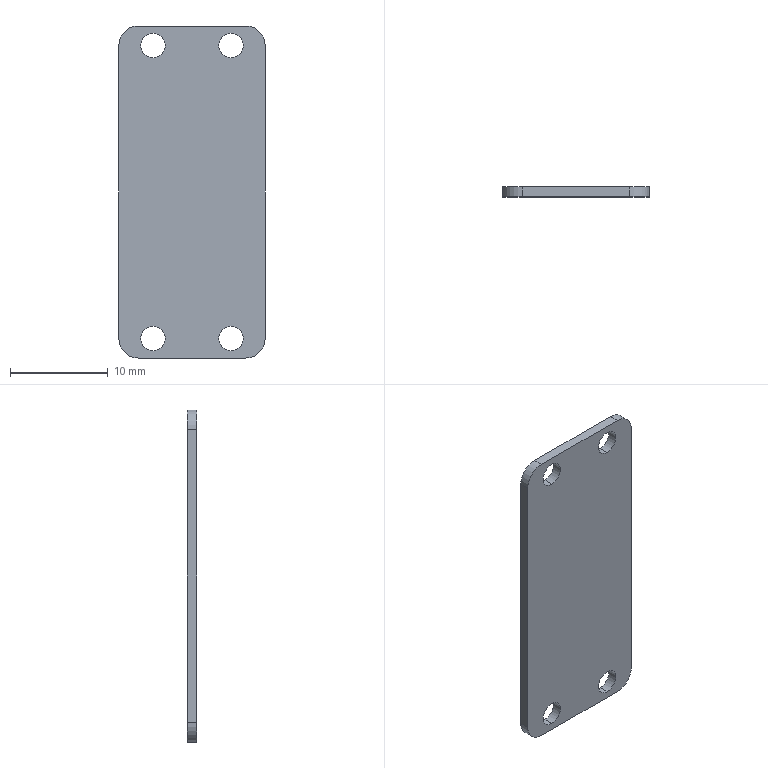CAM job | NX | mm | 3-axis | 1 set-up | 200 operations | part box 15 x 1 x 34
set-up 1
1. Cylinder Milling | Mill Mill5 LX-D1.5 | CYLINDER_MILLING_1 | path 297.004 mm | 0.1342 min
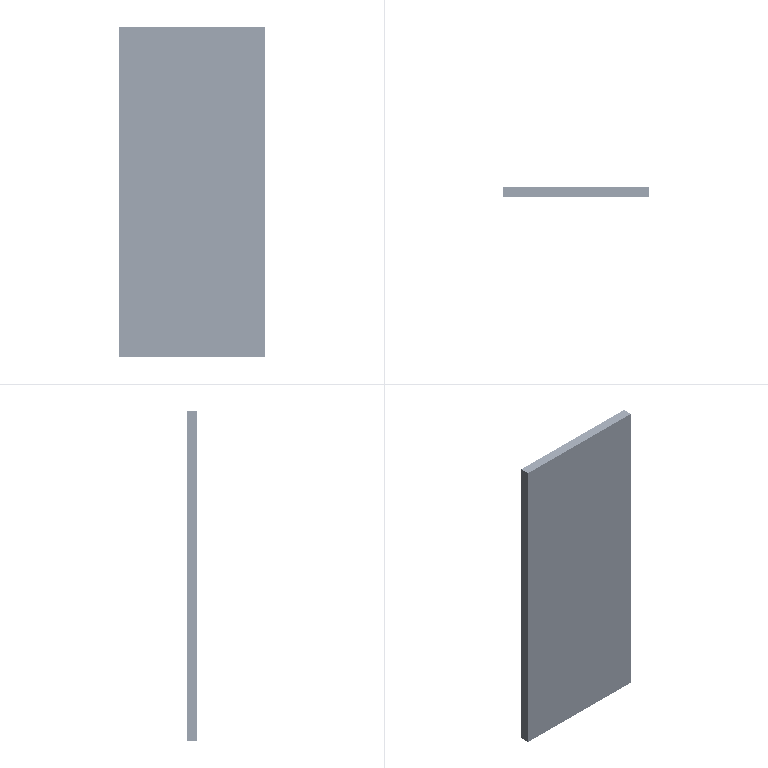2. Volume Based 2.5D Milling | Mill Mill5 LX-D1.5 | VOLUME_BASED_2.5D_MILLING_2 | path 646.751 mm | 0.2089 min
3. Cylinder Milling | Mill Mill5 LX-D1.5 | CYLINDER_MILLING_3 | path 297.004 mm | 0.1342 min
4. Volume Based 2.5D Milling | Mill Mill5 LX-D1.5 | VOLUME_BASED_2.5D_MILLING_4 | path 646.751 mm | 0.2089 min
5. Cylinder Milling | Mill Mill5 LX-D1.5 | CYLINDER_MILLING_5 | path 297.004 mm | 0.1342 min
6. Volume Based 2.5D Milling | Mill Mill5 LX-D1.5 | VOLUME_BASED_2.5D_MILLING_6 | path 646.751 mm | 0.2089 min
7. Cylinder Milling | Mill Mill5 LX-D1.5 | CYLINDER_MILLING_7 | path 297.004 mm | 0.1342 min
8. Volume Based 2.5D Milling | Mill Mill5 LX-D1.5 | VOLUME_BASED_2.5D_MILLING_8 | path 646.751 mm | 0.2089 min
9. Cylinder Milling | Mill Mill5 LX-D1.5 | CYLINDER_MILLING_9 | path 297.004 mm | 0.1342 min
10. Volume Based 2.5D Milling | Mill Mill5 LX-D1.5 | VOLUME_BASED_2.5D_MILLING_10 | path 646.751 mm | 0.2089 min
11. Cylinder Milling | Mill Mill5 LX-D1.5 | CYLINDER_MILLING_11 | path 297.004 mm | 0.1342 min
12. Volume Based 2.5D Milling | Mill Mill5 LX-D1.5 | VOLUME_BASED_2.5D_MILLING_12 | path 646.751 mm | 0.2089 min
13. Cylinder Milling | Mill Mill5 LX-D1.5 | CYLINDER_MILLING_13 | path 297.004 mm | 0.1342 min
14. Volume Based 2.5D Milling | Mill Mill5 LX-D1.5 | VOLUME_BASED_2.5D_MILLING_14 | path 646.751 mm | 0.2089 min
15. Cylinder Milling | Mill Mill5 LX-D1.5 | CYLINDER_MILLING_15 | path 297.004 mm | 0.1342 min
16. Volume Based 2.5D Milling | Mill Mill5 LX-D1.5 | VOLUME_BASED_2.5D_MILLING_16 | path 646.751 mm | 0.2089 min
17. Cylinder Milling | Mill Mill5 LX-D1.5 | CYLINDER_MILLING_17 | path 297.004 mm | 0.1342 min
18. Volume Based 2.5D Milling | Mill Mill5 LX-D1.5 | VOLUME_BASED_2.5D_MILLING_18 | path 646.751 mm | 0.2089 min
19. Cylinder Milling | Mill Mill5 LX-D1.5 | CYLINDER_MILLING_19 | path 297.004 mm | 0.1342 min
20. Volume Based 2.5D Milling | Mill Mill5 LX-D1.5 | VOLUME_BASED_2.5D_MILLING_20 | path 646.751 mm | 0.2089 min
21. Cylinder Milling | Mill Mill5 LX-D1.5 | CYLINDER_MILLING_21 | path 297.004 mm | 0.1342 min
22. Volume Based 2.5D Milling | Mill Mill5 LX-D1.5 | VOLUME_BASED_2.5D_MILLING_22 | path 646.751 mm | 0.2089 min
23. Cylinder Milling | Mill Mill5 LX-D1.5 | CYLINDER_MILLING_23 | path 297.004 mm | 0.1342 min
24. Volume Based 2.5D Milling | Mill Mill5 LX-D1.5 | VOLUME_BASED_2.5D_MILLING_24 | path 646.751 mm | 0.2089 min
25. Cylinder Milling | Mill Mill5 LX-D1.5 | CYLINDER_MILLING_25 | path 297.004 mm | 0.1342 min
26. Volume Based 2.5D Milling | Mill Mill5 LX-D1.5 | VOLUME_BASED_2.5D_MILLING_26 | path 646.751 mm | 0.2089 min
27. Cylinder Milling | Mill Mill5 LX-D1.5 | CYLINDER_MILLING_27 | path 297.004 mm | 0.1342 min
28. Volume Based 2.5D Milling | Mill Mill5 LX-D1.5 | VOLUME_BASED_2.5D_MILLING_28 | path 646.751 mm | 0.2089 min
29. Cylinder Milling | Mill Mill5 LX-D1.5 | CYLINDER_MILLING_29 | path 297.004 mm | 0.1342 min
30. Volume Based 2.5D Milling | Mill Mill5 LX-D1.5 | VOLUME_BASED_2.5D_MILLING_30 | path 646.751 mm | 0.2089 min
31. Cylinder Milling | Mill Mill5 LX-D1.5 | CYLINDER_MILLING_31 | path 297.004 mm | 0.1342 min
32. Volume Based 2.5D Milling | Mill Mill5 LX-D1.5 | VOLUME_BASED_2.5D_MILLING_32 | path 646.751 mm | 0.2089 min
33. Cylinder Milling | Mill Mill5 LX-D1.5 | CYLINDER_MILLING_33 | path 297.004 mm | 0.1342 min
34. Volume Based 2.5D Milling | Mill Mill5 LX-D1.5 | VOLUME_BASED_2.5D_MILLING_34 | path 646.751 mm | 0.2089 min
35. Cylinder Milling | Mill Mill5 LX-D1.5 | CYLINDER_MILLING_35 | path 297.004 mm | 0.1342 min
36. Volume Based 2.5D Milling | Mill Mill5 LX-D1.5 | VOLUME_BASED_2.5D_MILLING_36 | path 646.751 mm | 0.2089 min
37. Cylinder Milling | Mill Mill5 LX-D1.5 | CYLINDER_MILLING_37 | path 297.004 mm | 0.1342 min
38. Volume Based 2.5D Milling | Mill Mill5 LX-D1.5 | VOLUME_BASED_2.5D_MILLING_38 | path 646.751 mm | 0.2089 min
39. Cylinder Milling | Mill Mill5 LX-D1.5 | CYLINDER_MILLING_39 | path 297.004 mm | 0.1342 min
40. Volume Based 2.5D Milling | Mill Mill5 LX-D1.5 | VOLUME_BASED_2.5D_MILLING_40 | path 646.751 mm | 0.2089 min
41. Cylinder Milling | Mill Mill5 LX-D1.5 | CYLINDER_MILLING_41 | path 297.004 mm | 0.1342 min
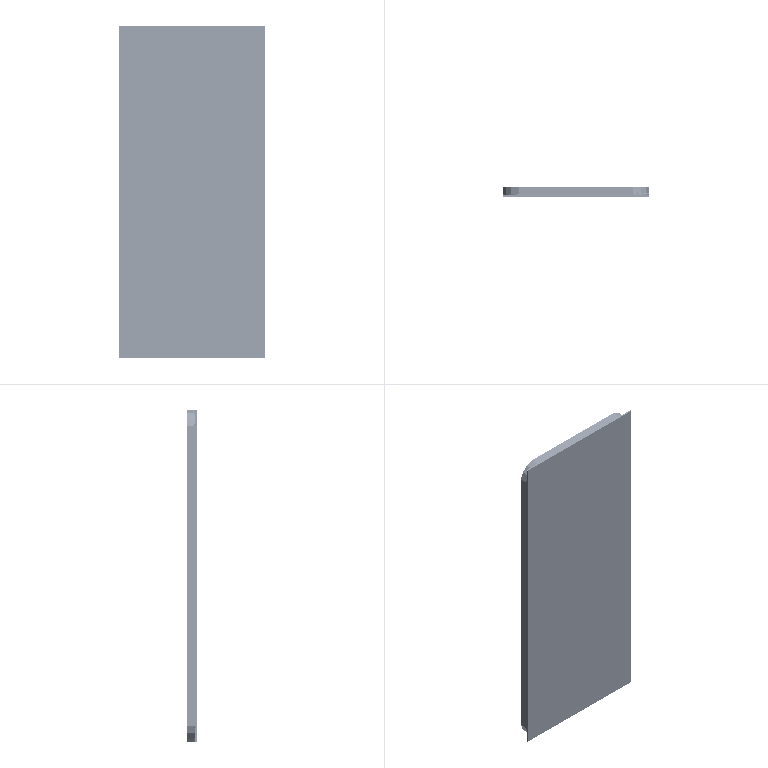42. Volume Based 2.5D Milling | Mill Mill5 LX-D1.5 | VOLUME_BASED_2.5D_MILLING_42 | path 646.751 mm | 0.2089 min
43. Cylinder Milling | Mill Mill5 LX-D1.5 | CYLINDER_MILLING_43 | path 297.004 mm | 0.1342 min
44. Volume Based 2.5D Milling | Mill Mill5 LX-D1.5 | VOLUME_BASED_2.5D_MILLING_44 | path 646.751 mm | 0.2089 min
45. Cylinder Milling | Mill Mill5 LX-D1.5 | CYLINDER_MILLING_45 | path 297.004 mm | 0.1342 min
46. Volume Based 2.5D Milling | Mill Mill5 LX-D1.5 | VOLUME_BASED_2.5D_MILLING_46 | path 646.751 mm | 0.2089 min
47. Cylinder Milling | Mill Mill5 LX-D1.5 | CYLINDER_MILLING_47 | path 297.004 mm | 0.1342 min
48. Volume Based 2.5D Milling | Mill Mill5 LX-D1.5 | VOLUME_BASED_2.5D_MILLING_48 | path 646.751 mm | 0.2089 min
49. Cylinder Milling | Mill Mill5 LX-D1.5 | CYLINDER_MILLING_49 | path 297.004 mm | 0.1342 min
50. Volume Based 2.5D Milling | Mill Mill5 LX-D1.5 | VOLUME_BASED_2.5D_MILLING_50 | path 646.751 mm | 0.2089 min
51. Cylinder Milling | Mill Mill5 LX-D1.5 | CYLINDER_MILLING_51 | path 297.004 mm | 0.1342 min
52. Volume Based 2.5D Milling | Mill Mill5 LX-D1.5 | VOLUME_BASED_2.5D_MILLING_52 | path 646.751 mm | 0.2089 min
53. Cylinder Milling | Mill Mill5 LX-D1.5 | CYLINDER_MILLING_53 | path 297.004 mm | 0.1342 min
54. Volume Based 2.5D Milling | Mill Mill5 LX-D1.5 | VOLUME_BASED_2.5D_MILLING_54 | path 646.751 mm | 0.2089 min
55. Cylinder Milling | Mill Mill5 LX-D1.5 | CYLINDER_MILLING_55 | path 297.004 mm | 0.1342 min
56. Volume Based 2.5D Milling | Mill Mill5 LX-D1.5 | VOLUME_BASED_2.5D_MILLING_56 | path 646.751 mm | 0.2089 min
57. Cylinder Milling | Mill Mill5 LX-D1.5 | CYLINDER_MILLING_57 | path 297.004 mm | 0.1342 min
58. Volume Based 2.5D Milling | Mill Mill5 LX-D1.5 | VOLUME_BASED_2.5D_MILLING_58 | path 646.751 mm | 0.2089 min
59. Cylinder Milling | Mill Mill5 LX-D1.5 | CYLINDER_MILLING_59 | path 297.004 mm | 0.1342 min
60. Volume Based 2.5D Milling | Mill Mill5 LX-D1.5 | VOLUME_BASED_2.5D_MILLING_60 | path 646.751 mm | 0.2089 min
61. Cylinder Milling | Mill Mill5 LX-D1.5 | CYLINDER_MILLING_61 | path 297.004 mm | 0.1342 min
62. Volume Based 2.5D Milling | Mill Mill5 LX-D1.5 | VOLUME_BASED_2.5D_MILLING_62 | path 646.751 mm | 0.2089 min
63. Cylinder Milling | Mill Mill5 LX-D1.5 | CYLINDER_MILLING_63 | path 297.004 mm | 0.1342 min
64. Volume Based 2.5D Milling | Mill Mill5 LX-D1.5 | VOLUME_BASED_2.5D_MILLING_64 | path 646.751 mm | 0.2089 min
65. Cylinder Milling | Mill Mill5 LX-D1.5 | CYLINDER_MILLING_65 | path 297.004 mm | 0.1342 min
66. Volume Based 2.5D Milling | Mill Mill5 LX-D1.5 | VOLUME_BASED_2.5D_MILLING_66 | path 646.751 mm | 0.2089 min
67. Cylinder Milling | Mill Mill5 LX-D1.5 | CYLINDER_MILLING_67 | path 297.004 mm | 0.1342 min
68. Volume Based 2.5D Milling | Mill Mill5 LX-D1.5 | VOLUME_BASED_2.5D_MILLING_68 | path 646.751 mm | 0.2089 min
69. Cylinder Milling | Mill Mill5 LX-D1.5 | CYLINDER_MILLING_69 | path 297.004 mm | 0.1342 min
70. Volume Based 2.5D Milling | Mill Mill5 LX-D1.5 | VOLUME_BASED_2.5D_MILLING_70 | path 646.751 mm | 0.2089 min
71. Cylinder Milling | Mill Mill5 LX-D1.5 | CYLINDER_MILLING_71 | path 297.004 mm | 0.1342 min
72. Volume Based 2.5D Milling | Mill Mill5 LX-D1.5 | VOLUME_BASED_2.5D_MILLING_72 | path 646.751 mm | 0.2089 min
73. Cylinder Milling | Mill Mill5 LX-D1.5 | CYLINDER_MILLING_73 | path 297.004 mm | 0.1342 min
74. Volume Based 2.5D Milling | Mill Mill5 LX-D1.5 | VOLUME_BASED_2.5D_MILLING_74 | path 646.751 mm | 0.2089 min
75. Cylinder Milling | Mill Mill5 LX-D1.5 | CYLINDER_MILLING_75 | path 297.004 mm | 0.1342 min
76. Volume Based 2.5D Milling | Mill Mill5 LX-D1.5 | VOLUME_BASED_2.5D_MILLING_76 | path 646.751 mm | 0.2089 min
77. Cylinder Milling | Mill Mill5 LX-D1.5 | CYLINDER_MILLING_77 | path 297.004 mm | 0.1342 min
78. Volume Based 2.5D Milling | Mill Mill5 LX-D1.5 | VOLUME_BASED_2.5D_MILLING_78 | path 646.751 mm | 0.2089 min
79. Cylinder Milling | Mill Mill5 LX-D1.5 | CYLINDER_MILLING_79 | path 297.004 mm | 0.1342 min
80. Volume Based 2.5D Milling | Mill Mill5 LX-D1.5 | VOLUME_BASED_2.5D_MILLING_80 | path 646.751 mm | 0.2089 min
81. Cylinder Milling | Mill Mill5 LX-D1.5 | CYLINDER_MILLING_81 | path 297.004 mm | 0.1342 min
82. Volume Based 2.5D Milling | Mill Mill5 LX-D1.5 | VOLUME_BASED_2.5D_MILLING_82 | path 646.751 mm | 0.2089 min
83. Cylinder Milling | Mill Mill5 LX-D1.5 | CYLINDER_MILLING_83 | path 297.004 mm | 0.1342 min
84. Volume Based 2.5D Milling | Mill Mill5 LX-D1.5 | VOLUME_BASED_2.5D_MILLING_84 | path 646.751 mm | 0.2089 min
85. Cylinder Milling | Mill Mill5 LX-D1.5 | CYLINDER_MILLING_85 | path 297.004 mm | 0.1342 min
86. Volume Based 2.5D Milling | Mill Mill5 LX-D1.5 | VOLUME_BASED_2.5D_MILLING_86 | path 646.751 mm | 0.2089 min
87. Cylinder Milling | Mill Mill5 LX-D1.5 | CYLINDER_MILLING_87 | path 297.004 mm | 0.1342 min
88. Volume Based 2.5D Milling | Mill Mill5 LX-D1.5 | VOLUME_BASED_2.5D_MILLING_88 | path 646.751 mm | 0.2089 min
89. Cylinder Milling | Mill Mill5 LX-D1.5 | CYLINDER_MILLING_89 | path 297.004 mm | 0.1342 min
90. Volume Based 2.5D Milling | Mill Mill5 LX-D1.5 | VOLUME_BASED_2.5D_MILLING_90 | path 646.751 mm | 0.2089 min
91. Cylinder Milling | Mill Mill5 LX-D1.5 | CYLINDER_MILLING_91 | path 297.004 mm | 0.1342 min
92. Volume Based 2.5D Milling | Mill Mill5 LX-D1.5 | VOLUME_BASED_2.5D_MILLING_92 | path 646.751 mm | 0.2089 min
93. Cylinder Milling | Mill Mill5 LX-D1.5 | CYLINDER_MILLING_93 | path 297.004 mm | 0.1342 min
94. Volume Based 2.5D Milling | Mill Mill5 LX-D1.5 | VOLUME_BASED_2.5D_MILLING_94 | path 646.751 mm | 0.2089 min
95. Cylinder Milling | Mill Mill5 LX-D1.5 | CYLINDER_MILLING_95 | path 297.004 mm | 0.1342 min
96. Volume Based 2.5D Milling | Mill Mill5 LX-D1.5 | VOLUME_BASED_2.5D_MILLING_96 | path 646.751 mm | 0.2089 min
97. Cylinder Milling | Mill Mill5 LX-D1.5 | CYLINDER_MILLING_97 | path 297.004 mm | 0.1342 min
98. Volume Based 2.5D Milling | Mill Mill5 LX-D1.5 | VOLUME_BASED_2.5D_MILLING_98 | path 646.751 mm | 0.2089 min
99. Cylinder Milling | Mill Mill5 LX-D1.5 | CYLINDER_MILLING_99 | path 297.004 mm | 0.1342 min
100. Volume Based 2.5D Milling | Mill Mill5 LX-D1.5 | VOLUME_BASED_2.5D_MILLING_100 | path 646.751 mm | 0.2089 min
101. Cylinder Milling | Mill Mill5 LX-D1.5J | CYLINDER_MILLING_101 | path 262.545 mm | 0.1627 min
102. Volume Based 2.5D Milling | Mill Mill5 LX-D1.5J | VOLUME_BASED_2.5D_MILLING_102 | path 142.793 mm | 0.1319 min
103. Cylinder Milling | Mill Mill5 LX-D1.5J | CYLINDER_MILLING_103 | path 262.545 mm | 0.1627 min
104. Volume Based 2.5D Milling | Mill Mill5 LX-D1.5J | VOLUME_BASED_2.5D_MILLING_104 | path 142.793 mm | 0.1319 min
105. Cylinder Milling | Mill Mill5 LX-D1.5J | CYLINDER_MILLING_105 | path 262.545 mm | 0.1627 min
106. Volume Based 2.5D Milling | Mill Mill5 LX-D1.5J | VOLUME_BASED_2.5D_MILLING_106 | path 142.793 mm | 0.1319 min
107. Cylinder Milling | Mill Mill5 LX-D1.5J | CYLINDER_MILLING_107 | path 262.545 mm | 0.1627 min
108. Volume Based 2.5D Milling | Mill Mill5 LX-D1.5J | VOLUME_BASED_2.5D_MILLING_108 | path 142.793 mm | 0.1319 min
109. Cylinder Milling | Mill Mill5 LX-D1.5J | CYLINDER_MILLING_109 | path 262.545 mm | 0.1627 min
110. Volume Based 2.5D Milling | Mill Mill5 LX-D1.5J | VOLUME_BASED_2.5D_MILLING_110 | path 142.793 mm | 0.1319 min
111. Cylinder Milling | Mill Mill5 LX-D1.5J | CYLINDER_MILLING_111 | path 262.545 mm | 0.1627 min
112. Volume Based 2.5D Milling | Mill Mill5 LX-D1.5J | VOLUME_BASED_2.5D_MILLING_112 | path 142.793 mm | 0.1319 min
113. Cylinder Milling | Mill Mill5 LX-D1.5J | CYLINDER_MILLING_113 | path 262.545 mm | 0.1627 min
114. Volume Based 2.5D Milling | Mill Mill5 LX-D1.5J | VOLUME_BASED_2.5D_MILLING_114 | path 142.793 mm | 0.1319 min
115. Cylinder Milling | Mill Mill5 LX-D1.5J | CYLINDER_MILLING_115 | path 262.545 mm | 0.1627 min
116. Volume Based 2.5D Milling | Mill Mill5 LX-D1.5J | VOLUME_BASED_2.5D_MILLING_116 | path 142.793 mm | 0.1319 min
117. Cylinder Milling | Mill Mill5 LX-D1.5J | CYLINDER_MILLING_117 | path 262.545 mm | 0.1627 min
118. Volume Based 2.5D Milling | Mill Mill5 LX-D1.5J | VOLUME_BASED_2.5D_MILLING_118 | path 142.793 mm | 0.1319 min
119. Cylinder Milling | Mill Mill5 LX-D1.5J | CYLINDER_MILLING_119 | path 262.545 mm | 0.1627 min
120. Volume Based 2.5D Milling | Mill Mill5 LX-D1.5J | VOLUME_BASED_2.5D_MILLING_120 | path 142.793 mm | 0.1319 min
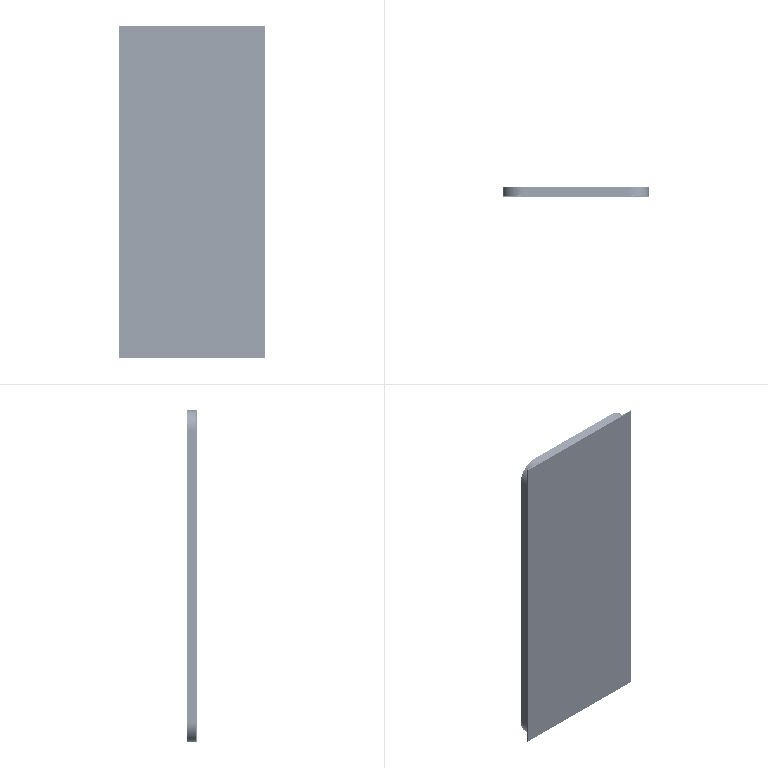121. Cylinder Milling | Mill Mill5 LX-D1.5J | CYLINDER_MILLING_121 | path 262.545 mm | 0.1627 min
122. Volume Based 2.5D Milling | Mill Mill5 LX-D1.5J | VOLUME_BASED_2.5D_MILLING_122 | path 142.793 mm | 0.1319 min
123. Cylinder Milling | Mill Mill5 LX-D1.5J | CYLINDER_MILLING_123 | path 262.545 mm | 0.1627 min
124. Volume Based 2.5D Milling | Mill Mill5 LX-D1.5J | VOLUME_BASED_2.5D_MILLING_124 | path 142.793 mm | 0.1319 min
125. Cylinder Milling | Mill Mill5 LX-D1.5J | CYLINDER_MILLING_125 | path 262.545 mm | 0.1627 min
126. Volume Based 2.5D Milling | Mill Mill5 LX-D1.5J | VOLUME_BASED_2.5D_MILLING_126 | path 142.793 mm | 0.1319 min
127. Cylinder Milling | Mill Mill5 LX-D1.5J | CYLINDER_MILLING_127 | path 262.545 mm | 0.1627 min
128. Volume Based 2.5D Milling | Mill Mill5 LX-D1.5J | VOLUME_BASED_2.5D_MILLING_128 | path 142.793 mm | 0.1319 min
129. Cylinder Milling | Mill Mill5 LX-D1.5J | CYLINDER_MILLING_129 | path 262.545 mm | 0.1627 min
130. Volume Based 2.5D Milling | Mill Mill5 LX-D1.5J | VOLUME_BASED_2.5D_MILLING_130 | path 142.793 mm | 0.1319 min
131. Cylinder Milling | Mill Mill5 LX-D1.5J | CYLINDER_MILLING_131 | path 262.545 mm | 0.1627 min
132. Volume Based 2.5D Milling | Mill Mill5 LX-D1.5J | VOLUME_BASED_2.5D_MILLING_132 | path 142.793 mm | 0.1319 min
133. Cylinder Milling | Mill Mill5 LX-D1.5J | CYLINDER_MILLING_133 | path 262.545 mm | 0.1627 min
134. Volume Based 2.5D Milling | Mill Mill5 LX-D1.5J | VOLUME_BASED_2.5D_MILLING_134 | path 142.793 mm | 0.1319 min
135. Cylinder Milling | Mill Mill5 LX-D1.5J | CYLINDER_MILLING_135 | path 262.545 mm | 0.1627 min
136. Volume Based 2.5D Milling | Mill Mill5 LX-D1.5J | VOLUME_BASED_2.5D_MILLING_136 | path 142.793 mm | 0.1319 min
137. Cylinder Milling | Mill Mill5 LX-D1.5J | CYLINDER_MILLING_137 | path 262.545 mm | 0.1627 min
138. Volume Based 2.5D Milling | Mill Mill5 LX-D1.5J | VOLUME_BASED_2.5D_MILLING_138 | path 142.793 mm | 0.1319 min
139. Cylinder Milling | Mill Mill5 LX-D1.5J | CYLINDER_MILLING_139 | path 262.545 mm | 0.1627 min
140. Volume Based 2.5D Milling | Mill Mill5 LX-D1.5J | VOLUME_BASED_2.5D_MILLING_140 | path 142.793 mm | 0.1319 min
141. Cylinder Milling | Mill Mill5 LX-D1.5J | CYLINDER_MILLING_141 | path 262.545 mm | 0.1627 min
142. Volume Based 2.5D Milling | Mill Mill5 LX-D1.5J | VOLUME_BASED_2.5D_MILLING_142 | path 142.793 mm | 0.1319 min
143. Cylinder Milling | Mill Mill5 LX-D1.5J | CYLINDER_MILLING_143 | path 262.545 mm | 0.1627 min
144. Volume Based 2.5D Milling | Mill Mill5 LX-D1.5J | VOLUME_BASED_2.5D_MILLING_144 | path 142.793 mm | 0.1319 min
145. Cylinder Milling | Mill Mill5 LX-D1.5J | CYLINDER_MILLING_145 | path 262.545 mm | 0.1627 min
146. Volume Based 2.5D Milling | Mill Mill5 LX-D1.5J | VOLUME_BASED_2.5D_MILLING_146 | path 142.793 mm | 0.1319 min
147. Cylinder Milling | Mill Mill5 LX-D1.5J | CYLINDER_MILLING_147 | path 262.545 mm | 0.1627 min
148. Volume Based 2.5D Milling | Mill Mill5 LX-D1.5J | VOLUME_BASED_2.5D_MILLING_148 | path 142.793 mm | 0.1319 min
149. Cylinder Milling | Mill Mill5 LX-D1.5J | CYLINDER_MILLING_149 | path 262.545 mm | 0.1627 min
150. Volume Based 2.5D Milling | Mill Mill5 LX-D1.5J | VOLUME_BASED_2.5D_MILLING_150 | path 142.793 mm | 0.1319 min
151. Cylinder Milling | Mill Mill5 LX-D1.5J | CYLINDER_MILLING_151 | path 262.545 mm | 0.1627 min
152. Volume Based 2.5D Milling | Mill Mill5 LX-D1.5J | VOLUME_BASED_2.5D_MILLING_152 | path 142.793 mm | 0.1319 min
153. Cylinder Milling | Mill Mill5 LX-D1.5J | CYLINDER_MILLING_153 | path 262.545 mm | 0.1627 min
154. Volume Based 2.5D Milling | Mill Mill5 LX-D1.5J | VOLUME_BASED_2.5D_MILLING_154 | path 142.793 mm | 0.1319 min
155. Cylinder Milling | Mill Mill5 LX-D1.5J | CYLINDER_MILLING_155 | path 262.545 mm | 0.1627 min
156. Volume Based 2.5D Milling | Mill Mill5 LX-D1.5J | VOLUME_BASED_2.5D_MILLING_156 | path 142.793 mm | 0.1319 min
157. Cylinder Milling | Mill Mill5 LX-D1.5J | CYLINDER_MILLING_157 | path 262.545 mm | 0.1627 min
158. Volume Based 2.5D Milling | Mill Mill5 LX-D1.5J | VOLUME_BASED_2.5D_MILLING_158 | path 142.793 mm | 0.1319 min
159. Cylinder Milling | Mill Mill5 LX-D1.5J | CYLINDER_MILLING_159 | path 262.545 mm | 0.1627 min
160. Volume Based 2.5D Milling | Mill Mill5 LX-D1.5J | VOLUME_BASED_2.5D_MILLING_160 | path 142.793 mm | 0.1319 min
161. Cylinder Milling | Mill Mill5 LX-D1.5J | CYLINDER_MILLING_161 | path 262.545 mm | 0.1627 min
162. Volume Based 2.5D Milling | Mill Mill5 LX-D1.5J | VOLUME_BASED_2.5D_MILLING_162 | path 142.793 mm | 0.1319 min
163. Cylinder Milling | Mill Mill5 LX-D1.5J | CYLINDER_MILLING_163 | path 262.545 mm | 0.1627 min
164. Volume Based 2.5D Milling | Mill Mill5 LX-D1.5J | VOLUME_BASED_2.5D_MILLING_164 | path 142.793 mm | 0.1319 min
165. Cylinder Milling | Mill Mill5 LX-D1.5J | CYLINDER_MILLING_165 | path 262.545 mm | 0.1627 min
166. Volume Based 2.5D Milling | Mill Mill5 LX-D1.5J | VOLUME_BASED_2.5D_MILLING_166 | path 142.793 mm | 0.1319 min
167. Cylinder Milling | Mill Mill5 LX-D1.5J | CYLINDER_MILLING_167 | path 262.545 mm | 0.1627 min
168. Volume Based 2.5D Milling | Mill Mill5 LX-D1.5J | VOLUME_BASED_2.5D_MILLING_168 | path 142.793 mm | 0.1319 min
169. Cylinder Milling | Mill Mill5 LX-D1.5J | CYLINDER_MILLING_169 | path 262.545 mm | 0.1627 min
170. Volume Based 2.5D Milling | Mill Mill5 LX-D1.5J | VOLUME_BASED_2.5D_MILLING_170 | path 142.793 mm | 0.1319 min
171. Cylinder Milling | Mill Mill5 LX-D1.5J | CYLINDER_MILLING_171 | path 262.545 mm | 0.1627 min
172. Volume Based 2.5D Milling | Mill Mill5 LX-D1.5J | VOLUME_BASED_2.5D_MILLING_172 | path 142.793 mm | 0.1319 min
173. Cylinder Milling | Mill Mill5 LX-D1.5J | CYLINDER_MILLING_173 | path 262.545 mm | 0.1627 min
174. Volume Based 2.5D Milling | Mill Mill5 LX-D1.5J | VOLUME_BASED_2.5D_MILLING_174 | path 142.793 mm | 0.1319 min
175. Cylinder Milling | Mill Mill5 LX-D1.5J | CYLINDER_MILLING_175 | path 262.545 mm | 0.1627 min
176. Volume Based 2.5D Milling | Mill Mill5 LX-D1.5J | VOLUME_BASED_2.5D_MILLING_176 | path 142.793 mm | 0.1319 min
177. Cylinder Milling | Mill Mill5 LX-D1.5J | CYLINDER_MILLING_177 | path 262.545 mm | 0.1627 min
178. Volume Based 2.5D Milling | Mill Mill5 LX-D1.5J | VOLUME_BASED_2.5D_MILLING_178 | path 142.793 mm | 0.1319 min
179. Cylinder Milling | Mill Mill5 LX-D1.5J | CYLINDER_MILLING_179 | path 262.545 mm | 0.1627 min
180. Volume Based 2.5D Milling | Mill Mill5 LX-D1.5J | VOLUME_BASED_2.5D_MILLING_180 | path 142.793 mm | 0.1319 min
181. Cylinder Milling | Mill Mill5 LX-D1.5J | CYLINDER_MILLING_181 | path 262.545 mm | 0.1627 min
182. Volume Based 2.5D Milling | Mill Mill5 LX-D1.5J | VOLUME_BASED_2.5D_MILLING_182 | path 142.793 mm | 0.1319 min
183. Cylinder Milling | Mill Mill5 LX-D1.5J | CYLINDER_MILLING_183 | path 262.545 mm | 0.1627 min
184. Volume Based 2.5D Milling | Mill Mill5 LX-D1.5J | VOLUME_BASED_2.5D_MILLING_184 | path 142.793 mm | 0.1319 min
185. Cylinder Milling | Mill Mill5 LX-D1.5J | CYLINDER_MILLING_185 | path 262.545 mm | 0.1627 min
186. Volume Based 2.5D Milling | Mill Mill5 LX-D1.5J | VOLUME_BASED_2.5D_MILLING_186 | path 142.793 mm | 0.1319 min
187. Cylinder Milling | Mill Mill5 LX-D1.5J | CYLINDER_MILLING_187 | path 262.545 mm | 0.1627 min
188. Volume Based 2.5D Milling | Mill Mill5 LX-D1.5J | VOLUME_BASED_2.5D_MILLING_188 | path 142.793 mm | 0.1319 min
189. Cylinder Milling | Mill Mill5 LX-D1.5J | CYLINDER_MILLING_189 | path 262.545 mm | 0.1627 min
190. Volume Based 2.5D Milling | Mill Mill5 LX-D1.5J | VOLUME_BASED_2.5D_MILLING_190 | path 142.793 mm | 0.1319 min
191. Cylinder Milling | Mill Mill5 LX-D1.5J | CYLINDER_MILLING_191 | path 262.545 mm | 0.1627 min
192. Volume Based 2.5D Milling | Mill Mill5 LX-D1.5J | VOLUME_BASED_2.5D_MILLING_192 | path 142.793 mm | 0.1319 min
193. Cylinder Milling | Mill Mill5 LX-D1.5J | CYLINDER_MILLING_193 | path 262.545 mm | 0.1627 min
194. Volume Based 2.5D Milling | Mill Mill5 LX-D1.5J | VOLUME_BASED_2.5D_MILLING_194 | path 142.793 mm | 0.1319 min
195. Cylinder Milling | Mill Mill5 LX-D1.5J | CYLINDER_MILLING_195 | path 262.545 mm | 0.1627 min
196. Volume Based 2.5D Milling | Mill Mill5 LX-D1.5J | VOLUME_BASED_2.5D_MILLING_196 | path 142.793 mm | 0.1319 min
197. Cylinder Milling | Mill Mill5 LX-D1.5J | CYLINDER_MILLING_197 | path 262.545 mm | 0.1627 min
198. Volume Based 2.5D Milling | Mill Mill5 LX-D1.5J | VOLUME_BASED_2.5D_MILLING_198 | path 142.793 mm | 0.1319 min
199. Cylinder Milling | Mill Mill5 LX-D1.5J | CYLINDER_MILLING_199 | path 262.545 mm | 0.1627 min
200. Volume Based 2.5D Milling | Mill Mill5 LX-D1.5J | VOLUME_BASED_2.5D_MILLING_200 | path 142.793 mm | 0.1319 min